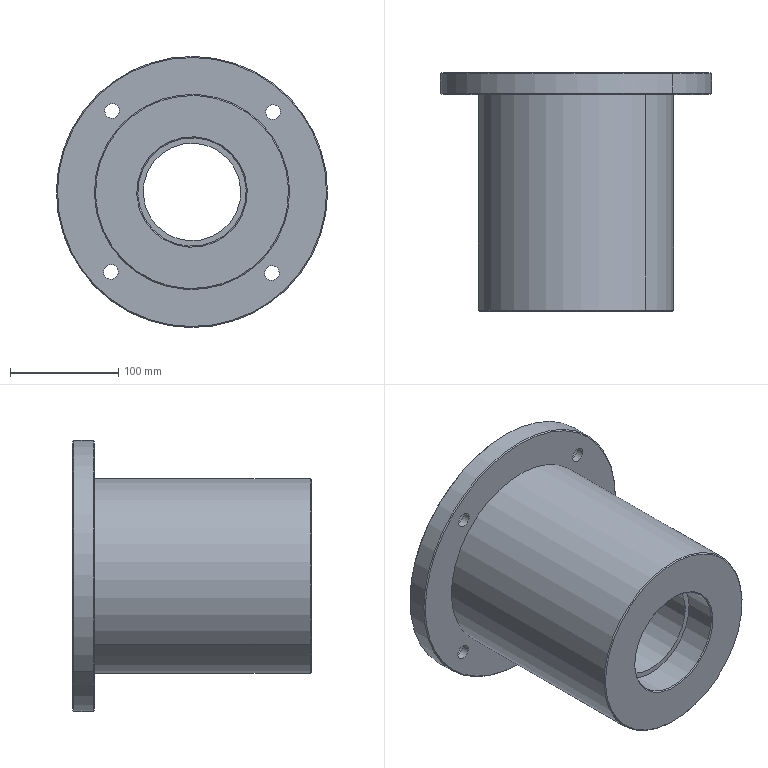Component | SolidWorks | 008A-20130717-1 | 1 solid | 48 faces | volume 3727844 mm3 | cylinder 28 | cone 10 | plane 10 | commonest cylinder face diameters 20 x8 13.5 x8 130 x2 100 x2 150 x2 180 x2 250 x2 90 x2